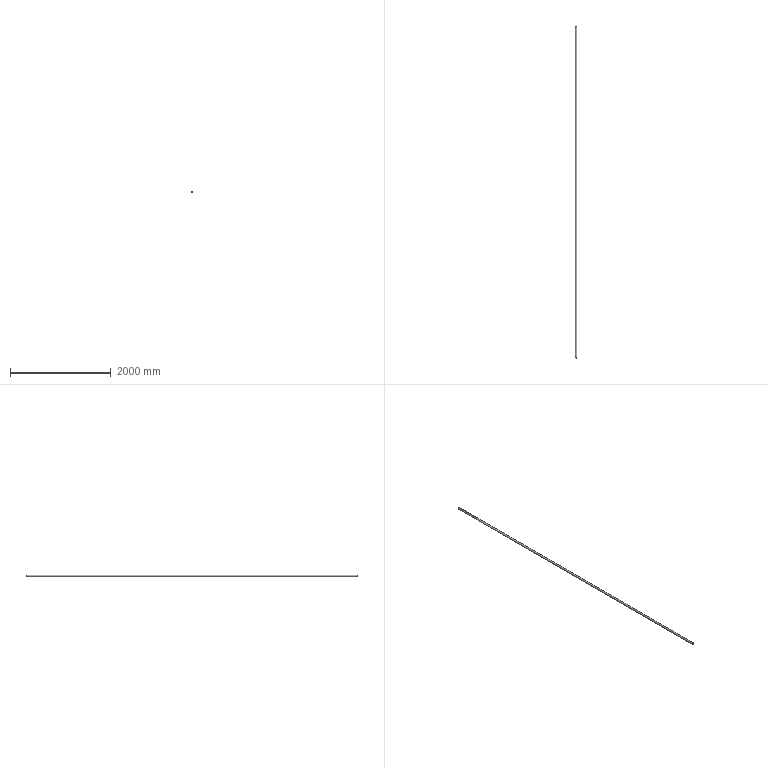Component | NX | 43_4 | 1 solid | 4 faces | volume 2213074 mm3 | cylinder 2 | plane 2 | commonest cylinder face diameters 34 x1 27 x1